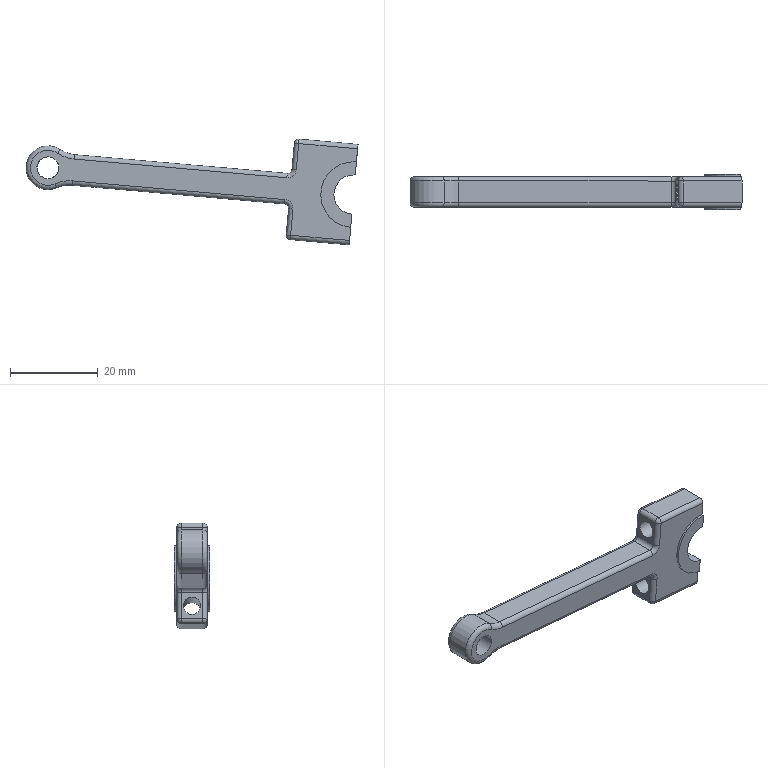Component | NX | CONNECTING_ROD_1 | 1 solid | 51 faces | volume 4645 mm3 | cylinder 25 | plane 12 | torus 10 | sphere 4 | commonest cylinder face diameters 2 x16 15 x2 14 x2 4 x2 10 x1 9 x1 5 x1